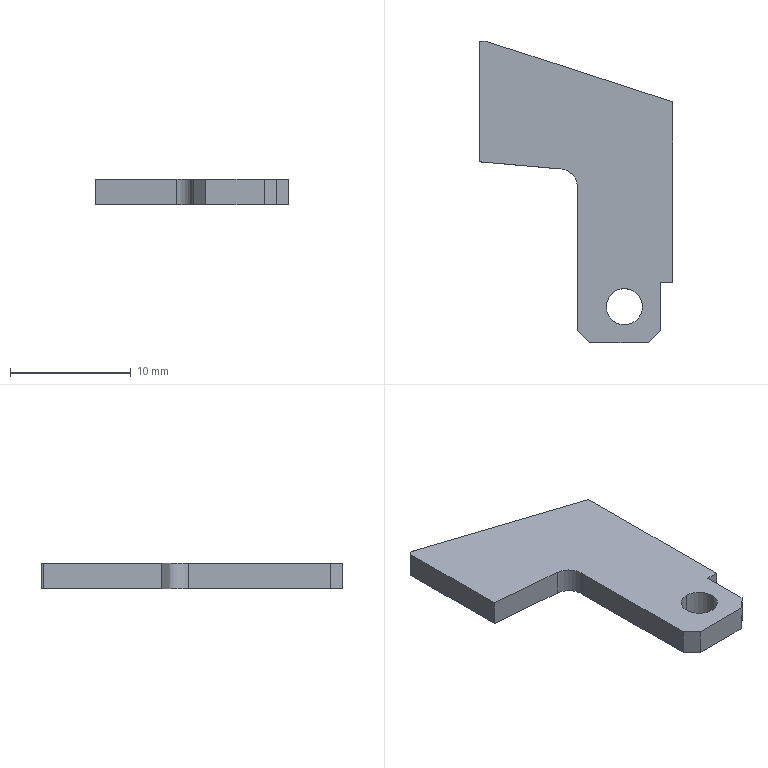Component | SolidWorks | 17268061-1 | 1 solid | 18 faces | box 16 x 25 x 2.1 mm | volume 482 mm3 | plane 13 | cylinder 5 | commonest cylinder face diameters 3 x3 0.4 x2 | material SKD-11 HRC58° Electroplated
STEP:
#1=CARTESIAN_POINT('',(2.264,-1.027,-0.3346));
#2=VERTEX_POINT('',#1);
#3=CARTESIAN_POINT('',(2.264,-1.145,-0.3346));
#4=VERTEX_POINT('',#3);
#5=CARTESIAN_POINT('',(2.264,-1.086,-0.3346));
#6=DIRECTION('',(-0.,0.,-1.));
#7=DIRECTION('',(0.,-1.,-0.));
#8=AXIS2_PLACEMENT_3D('',#5,#6,#7);
#9=CIRCLE('',#8,0.05906);
#10=EDGE_CURVE('',#2,#4,#9,.T.);
#11=ORIENTED_EDGE('',*,*,#10,.F.);
#12=CARTESIAN_POINT('',(2.264,-1.027,-0.4173));
#13=VERTEX_POINT('',#12);
#14=CARTESIAN_POINT('',(2.264,-1.027,-0.3346));
#15=DIRECTION('',(-0.,0.,-1.));
#16=VECTOR('',#15,39.37);
#17=LINE('',#14,#16);
#18=EDGE_CURVE('',#2,#13,#17,.T.);
#19=ORIENTED_EDGE('',*,*,#18,.T.);
#20=CARTESIAN_POINT('',(2.264,-1.145,-0.4173));
#21=VERTEX_POINT('',#20);
#22=CARTESIAN_POINT('',(2.264,-1.086,-0.4173));
#23=DIRECTION('',(-0.,0.,-1.));
#24=DIRECTION('',(0.,-1.,-0.));
#25=AXIS2_PLACEMENT_3D('',#22,#23,#24);
#26=CIRCLE('',#25,0.05906);
#27=EDGE_CURVE('',#13,#21,#26,.T.);
#28=ORIENTED_EDGE('',*,*,#27,.T.);
#29=CARTESIAN_POINT('',(2.264,-1.145,-0.3346));
#30=DIRECTION('',(-0.,0.,-1.));
#31=VECTOR('',#30,39.37);
#32=LINE('',#29,#31);
#33=EDGE_CURVE('',#4,#21,#32,.T.);
#34=ORIENTED_EDGE('',*,*,#33,.F.);
#35=EDGE_LOOP('',(#11,#19,#28,#34));
#36=FACE_OUTER_BOUND('',#35,.T.);
#37=CARTESIAN_POINT('',(2.264,-1.086,-0.3346));
#38=DIRECTION('',(-0.,0.,-1.));
#39=DIRECTION('',(0.,-1.,-0.));
#40=AXIS2_PLACEMENT_3D('',#37,#38,#39);
#41=CYLINDRICAL_SURFACE('',#40,0.05906);
#42=ADVANCED_FACE('',(#36),#41,.F.);
#43=CARTESIAN_POINT('',(2.421,-0.4179,-0.3346));
#44=VERTEX_POINT('',#43);
#45=CARTESIAN_POINT('',(2.421,-1.007,-0.3346));
#46=VERTEX_POINT('',#45);
#47=CARTESIAN_POINT('',(2.421,-0.2197,-0.3346));
#48=DIRECTION('',(-0.,-1.,-0.));
#49=VECTOR('',#48,39.37);
#50=LINE('',#47,#49);
#51=EDGE_CURVE('',#44,#46,#50,.T.);
#52=ORIENTED_EDGE('',*,*,#51,.T.);
#53=CARTESIAN_POINT('',(2.421,-1.007,-0.4173));
#54=VERTEX_POINT('',#53);
#55=CARTESIAN_POINT('',(2.421,-1.007,-0.3346));
#56=DIRECTION('',(-0.,0.,-1.));
#57=VECTOR('',#56,39.37);
#58=LINE('',#55,#57);
#59=EDGE_CURVE('',#46,#54,#58,.T.);
#60=ORIENTED_EDGE('',*,*,#59,.T.);
#61=CARTESIAN_POINT('',(2.421,-0.4179,-0.4173));
#62=VERTEX_POINT('',#61);
#63=CARTESIAN_POINT('',(2.421,-0.2197,-0.4173));
#64=DIRECTION('',(-0.,-1.,-0.));
#65=VECTOR('',#64,39.37);
#66=LINE('',#63,#65);
#67=EDGE_CURVE('',#62,#54,#66,.T.);
#68=ORIENTED_EDGE('',*,*,#67,.F.);
#69=CARTESIAN_POINT('',(2.421,-0.4179,-0.4173));
#70=DIRECTION('',(0.,-0.,1.));
#71=VECTOR('',#70,39.37);
#72=LINE('',#69,#71);
#73=EDGE_CURVE('',#62,#44,#72,.T.);
#74=ORIENTED_EDGE('',*,*,#73,.T.);
#75=EDGE_LOOP('',(#52,#60,#68,#74));
#76=FACE_OUTER_BOUND('',#75,.T.);
#77=CARTESIAN_POINT('',(2.421,-0.2197,-0.4173));
#78=DIRECTION('',(-1.,0.,0.));
#79=DIRECTION('',(0.,1.,0.));
#80=AXIS2_PLACEMENT_3D('',#77,#78,#79);
#81=PLANE('',#80);
#82=ADVANCED_FACE('',(#76),#81,.F.);
#83=CARTESIAN_POINT('',(2.343,-1.204,-0.3346));
#84=VERTEX_POINT('',#83);
#85=CARTESIAN_POINT('',(2.15,-1.204,-0.3346));
#86=VERTEX_POINT('',#85);
#87=CARTESIAN_POINT('',(2.421,-1.204,-0.3346));
#88=DIRECTION('',(-1.,0.,0.));
#89=VECTOR('',#88,39.37);
#90=LINE('',#87,#89);
#91=EDGE_CURVE('',#84,#86,#90,.T.);
#92=ORIENTED_EDGE('',*,*,#91,.T.);
#93=CARTESIAN_POINT('',(2.15,-1.204,-0.4173));
#94=VERTEX_POINT('',#93);
#95=CARTESIAN_POINT('',(2.15,-1.204,-0.4173));
#96=DIRECTION('',(-0.,0.,-1.));
#97=VECTOR('',#96,39.37);
#98=LINE('',#95,#97);
#99=EDGE_CURVE('',#86,#94,#98,.T.);
#100=ORIENTED_EDGE('',*,*,#99,.T.);
#101=CARTESIAN_POINT('',(2.343,-1.204,-0.4173));
#102=VERTEX_POINT('',#101);
#103=CARTESIAN_POINT('',(2.421,-1.204,-0.4173));
#104=DIRECTION('',(-1.,0.,0.));
#105=VECTOR('',#104,39.37);
#106=LINE('',#103,#105);
#107=EDGE_CURVE('',#102,#94,#106,.T.);
#108=ORIENTED_EDGE('',*,*,#107,.F.);
#109=CARTESIAN_POINT('',(2.343,-1.204,-0.4173));
#110=DIRECTION('',(0.,-0.,1.));
#111=VECTOR('',#110,39.37);
#112=LINE('',#109,#111);
#113=EDGE_CURVE('',#102,#84,#112,.T.);
#114=ORIENTED_EDGE('',*,*,#113,.T.);
#115=EDGE_LOOP('',(#92,#100,#108,#114));
#116=FACE_OUTER_BOUND('',#115,.T.);
#117=CARTESIAN_POINT('',(2.421,-1.204,-0.4173));
#118=DIRECTION('',(0.,1.,0.));
#119=DIRECTION('',(1.,-0.,-0.));
#120=AXIS2_PLACEMENT_3D('',#117,#118,#119);
#121=PLANE('',#120);
#122=ADVANCED_FACE('',(#116),#121,.F.);
#123=CARTESIAN_POINT('',(1.791,-0.6134,-0.3346));
#124=VERTEX_POINT('',#123);
#125=CARTESIAN_POINT('',(1.791,-0.2275,-0.3346));
#126=VERTEX_POINT('',#125);
#127=CARTESIAN_POINT('',(1.791,-0.2197,-0.3346));
#128=DIRECTION('',(0.,1.,0.));
#129=VECTOR('',#128,39.37);
#130=LINE('',#127,#129);
#131=EDGE_CURVE('',#124,#126,#130,.T.);
#132=ORIENTED_EDGE('',*,*,#131,.T.);
#133=CARTESIAN_POINT('',(1.791,-0.2275,-0.4173));
#134=VERTEX_POINT('',#133);
#135=CARTESIAN_POINT('',(1.791,-0.2275,-0.4173));
#136=DIRECTION('',(-0.,0.,-1.));
#137=VECTOR('',#136,39.37);
#138=LINE('',#135,#137);
#139=EDGE_CURVE('',#126,#134,#138,.T.);
#140=ORIENTED_EDGE('',*,*,#139,.T.);
#141=CARTESIAN_POINT('',(1.791,-0.6134,-0.4173));
#142=VERTEX_POINT('',#141);
#143=CARTESIAN_POINT('',(1.791,-0.2197,-0.4173));
#144=DIRECTION('',(0.,1.,0.));
#145=VECTOR('',#144,39.37);
#146=LINE('',#143,#145);
#147=EDGE_CURVE('',#142,#134,#146,.T.);
#148=ORIENTED_EDGE('',*,*,#147,.F.);
#149=CARTESIAN_POINT('',(1.791,-0.6134,-0.3346));
#150=DIRECTION('',(-0.,0.,-1.));
#151=VECTOR('',#150,39.37);
#152=LINE('',#149,#151);
#153=EDGE_CURVE('',#124,#142,#152,.T.);
#154=ORIENTED_EDGE('',*,*,#153,.F.);
#155=EDGE_LOOP('',(#132,#140,#148,#154));
#156=FACE_OUTER_BOUND('',#155,.T.);
#157=CARTESIAN_POINT('',(1.791,-0.2197,-0.4173));
#158=DIRECTION('',(1.,-0.,-0.));
#159=DIRECTION('',(-0.,-1.,-0.));
#160=AXIS2_PLACEMENT_3D('',#157,#158,#159);
#161=PLANE('',#160);
#162=ADVANCED_FACE('',(#156),#161,.F.);
#163=CARTESIAN_POINT('',(1.799,-0.2197,-0.3346));
#164=VERTEX_POINT('',#163);
#165=CARTESIAN_POINT('',(1.81,-0.2197,-0.3346));
#166=VERTEX_POINT('',#165);
#167=CARTESIAN_POINT('',(2.421,-0.2197,-0.3346));
#168=DIRECTION('',(1.,-0.,-0.));
#169=VECTOR('',#168,39.37);
#170=LINE('',#167,#169);
#171=EDGE_CURVE('',#164,#166,#170,.T.);
#172=ORIENTED_EDGE('',*,*,#171,.T.);
#173=CARTESIAN_POINT('',(1.81,-0.2197,-0.4173));
#174=VERTEX_POINT('',#173);
#175=CARTESIAN_POINT('',(1.81,-0.2197,-0.4173));
#176=DIRECTION('',(-0.,0.,-1.));
#177=VECTOR('',#176,39.37);
#178=LINE('',#175,#177);
#179=EDGE_CURVE('',#166,#174,#178,.T.);
#180=ORIENTED_EDGE('',*,*,#179,.T.);
#181=CARTESIAN_POINT('',(1.799,-0.2197,-0.4173));
#182=VERTEX_POINT('',#181);
#183=CARTESIAN_POINT('',(2.421,-0.2197,-0.4173));
#184=DIRECTION('',(1.,-0.,-0.));
#185=VECTOR('',#184,39.37);
#186=LINE('',#183,#185);
#187=EDGE_CURVE('',#182,#174,#186,.T.);
#188=ORIENTED_EDGE('',*,*,#187,.F.);
#189=CARTESIAN_POINT('',(1.799,-0.2197,-0.4173));
#190=DIRECTION('',(0.,-0.,1.));
#191=VECTOR('',#190,39.37);
#192=LINE('',#189,#191);
#193=EDGE_CURVE('',#182,#164,#192,.T.);
#194=ORIENTED_EDGE('',*,*,#193,.T.);
#195=EDGE_LOOP('',(#172,#180,#188,#194));
#196=FACE_OUTER_BOUND('',#195,.T.);
#197=CARTESIAN_POINT('',(2.421,-0.2197,-0.4173));
#198=DIRECTION('',(-0.,-1.,-0.));
#199=DIRECTION('',(-1.,0.,0.));
#200=AXIS2_PLACEMENT_3D('',#197,#198,#199);
#201=PLANE('',#200);
#202=ADVANCED_FACE('',(#196),#201,.F.);
#203=ORIENTED_EDGE('',*,*,#107,.T.);
#204=CARTESIAN_POINT('',(2.111,-1.165,-0.4173));
#205=VERTEX_POINT('',#204);
#206=CARTESIAN_POINT('',(2.286,-1.339,-0.4173));
#207=DIRECTION('',(-0.7071,0.7071,0.));
#208=VECTOR('',#207,39.37);
#209=LINE('',#206,#208);
#210=EDGE_CURVE('',#94,#205,#209,.T.);
#211=ORIENTED_EDGE('',*,*,#210,.T.);
#212=CARTESIAN_POINT('',(2.111,-0.7006,-0.4173));
#213=VERTEX_POINT('',#212);
#214=CARTESIAN_POINT('',(2.111,-0.7006,-0.4173));
#215=DIRECTION('',(-0.,-1.,-0.));
#216=VECTOR('',#215,39.37);
#217=LINE('',#214,#216);
#218=EDGE_CURVE('',#213,#205,#217,.T.);
#219=ORIENTED_EDGE('',*,*,#218,.F.);
#220=CARTESIAN_POINT('',(2.057,-0.6366,-0.4173));
#221=VERTEX_POINT('',#220);
#222=CARTESIAN_POINT('',(2.052,-0.6955,-0.4173));
#223=DIRECTION('',(0.,-0.,1.));
#224=DIRECTION('',(0.,-1.,-0.));
#225=AXIS2_PLACEMENT_3D('',#222,#223,#224);
#226=CIRCLE('',#225,0.05906);
#227=EDGE_CURVE('',#213,#221,#226,.T.);
#228=ORIENTED_EDGE('',*,*,#227,.T.);
#229=CARTESIAN_POINT('',(1.791,-0.6134,-0.4173));
#230=DIRECTION('',(0.9962,-0.08716,-0.));
#231=VECTOR('',#230,39.37);
#232=LINE('',#229,#231);
#233=EDGE_CURVE('',#142,#221,#232,.T.);
#234=ORIENTED_EDGE('',*,*,#233,.F.);
#235=ORIENTED_EDGE('',*,*,#147,.T.);
#236=CARTESIAN_POINT('',(1.799,-0.2275,-0.4173));
#237=DIRECTION('',(-0.,0.,-1.));
#238=DIRECTION('',(0.,-1.,0.));
#239=AXIS2_PLACEMENT_3D('',#236,#237,#238);
#240=CIRCLE('',#239,0.007874);
#241=EDGE_CURVE('',#134,#182,#240,.T.);
#242=ORIENTED_EDGE('',*,*,#241,.T.);
#243=ORIENTED_EDGE('',*,*,#187,.T.);
#244=CARTESIAN_POINT('',(1.812,-0.22,-0.4173));
#245=VERTEX_POINT('',#244);
#246=CARTESIAN_POINT('',(1.81,-0.2275,-0.4173));
#247=DIRECTION('',(-0.,0.,-1.));
#248=DIRECTION('',(0.,-1.,0.));
#249=AXIS2_PLACEMENT_3D('',#246,#247,#248);
#250=CIRCLE('',#249,0.007874);
#251=EDGE_CURVE('',#174,#245,#250,.T.);
#252=ORIENTED_EDGE('',*,*,#251,.T.);
#253=CARTESIAN_POINT('',(2.421,-0.4179,-0.4173));
#254=DIRECTION('',(0.9511,-0.309,-0.));
#255=VECTOR('',#254,39.37);
#256=LINE('',#253,#255);
#257=EDGE_CURVE('',#245,#62,#256,.T.);
#258=ORIENTED_EDGE('',*,*,#257,.T.);
#259=ORIENTED_EDGE('',*,*,#67,.T.);
#260=CARTESIAN_POINT('',(2.382,-1.007,-0.4173));
#261=VERTEX_POINT('',#260);
#262=CARTESIAN_POINT('',(2.421,-1.007,-0.4173));
#263=DIRECTION('',(1.,-0.,-0.));
#264=VECTOR('',#263,39.37);
#265=LINE('',#262,#264);
#266=EDGE_CURVE('',#261,#54,#265,.T.);
#267=ORIENTED_EDGE('',*,*,#266,.F.);
#268=CARTESIAN_POINT('',(2.382,-1.165,-0.4173));
#269=VERTEX_POINT('',#268);
#270=CARTESIAN_POINT('',(2.382,-1.007,-0.4173));
#271=DIRECTION('',(0.,1.,0.));
#272=VECTOR('',#271,39.37);
#273=LINE('',#270,#272);
#274=EDGE_CURVE('',#269,#261,#273,.T.);
#275=ORIENTED_EDGE('',*,*,#274,.F.);
#276=CARTESIAN_POINT('',(2.382,-1.165,-0.4173));
#277=DIRECTION('',(-0.7071,-0.7071,0.));
#278=VECTOR('',#277,39.37);
#279=LINE('',#276,#278);
#280=EDGE_CURVE('',#269,#102,#279,.T.);
#281=ORIENTED_EDGE('',*,*,#280,.T.);
#282=EDGE_LOOP('',(#203,#211,#219,#228,#234,#235,#242,#243,#252,#258,#259,#267,#275,#281));
#283=FACE_OUTER_BOUND('',#282,.T.);
#284=CARTESIAN_POINT('',(2.264,-1.086,-0.4173));
#285=DIRECTION('',(-0.,0.,-1.));
#286=DIRECTION('',(0.,-1.,-0.));
#287=AXIS2_PLACEMENT_3D('',#284,#285,#286);
#288=CIRCLE('',#287,0.05906);
#289=EDGE_CURVE('',#21,#13,#288,.T.);
#290=ORIENTED_EDGE('',*,*,#289,.F.);
#291=ORIENTED_EDGE('',*,*,#27,.F.);
#292=EDGE_LOOP('',(#290,#291));
#293=FACE_BOUND('',#292,.T.);
#294=CARTESIAN_POINT('',(2.421,-1.204,-0.4173));
#295=DIRECTION('',(-0.,0.,-1.));
#296=DIRECTION('',(-0.,-1.,-0.));
#297=AXIS2_PLACEMENT_3D('',#294,#295,#296);
#298=PLANE('',#297);
#299=ADVANCED_FACE('',(#283,#293),#298,.T.);
#300=CARTESIAN_POINT('',(2.264,-1.086,-0.3346));
#301=DIRECTION('',(-0.,0.,-1.));
#302=DIRECTION('',(0.,-1.,-0.));
#303=AXIS2_PLACEMENT_3D('',#300,#301,#302);
#304=CIRCLE('',#303,0.05906);
#305=EDGE_CURVE('',#4,#2,#304,.T.);
#306=ORIENTED_EDGE('',*,*,#305,.T.);
#307=ORIENTED_EDGE('',*,*,#10,.T.);
#308=EDGE_LOOP('',(#306,#307));
#309=FACE_BOUND('',#308,.T.);
#310=CARTESIAN_POINT('',(2.111,-0.7006,-0.3346));
#311=VERTEX_POINT('',#310);
#312=CARTESIAN_POINT('',(2.111,-1.165,-0.3346));
#313=VERTEX_POINT('',#312);
#314=CARTESIAN_POINT('',(2.111,-0.7006,-0.3346));
#315=DIRECTION('',(-0.,-1.,-0.));
#316=VECTOR('',#315,39.37);
#317=LINE('',#314,#316);
#318=EDGE_CURVE('',#311,#313,#317,.T.);
#319=ORIENTED_EDGE('',*,*,#318,.T.);
#320=CARTESIAN_POINT('',(2.15,-1.204,-0.3346));
#321=DIRECTION('',(0.7071,-0.7071,-0.));
#322=VECTOR('',#321,39.37);
#323=LINE('',#320,#322);
#324=EDGE_CURVE('',#313,#86,#323,.T.);
#325=ORIENTED_EDGE('',*,*,#324,.T.);
#326=ORIENTED_EDGE('',*,*,#91,.F.);
#327=CARTESIAN_POINT('',(2.382,-1.165,-0.3346));
#328=VERTEX_POINT('',#327);
#329=CARTESIAN_POINT('',(2.382,-1.165,-0.3346));
#330=DIRECTION('',(0.7071,0.7071,-0.));
#331=VECTOR('',#330,39.37);
#332=LINE('',#329,#331);
#333=EDGE_CURVE('',#84,#328,#332,.T.);
#334=ORIENTED_EDGE('',*,*,#333,.T.);
#335=CARTESIAN_POINT('',(2.382,-1.007,-0.3346));
#336=VERTEX_POINT('',#335);
#337=CARTESIAN_POINT('',(2.382,-1.007,-0.3346));
#338=DIRECTION('',(0.,1.,0.));
#339=VECTOR('',#338,39.37);
#340=LINE('',#337,#339);
#341=EDGE_CURVE('',#328,#336,#340,.T.);
#342=ORIENTED_EDGE('',*,*,#341,.T.);
#343=CARTESIAN_POINT('',(2.421,-1.007,-0.3346));
#344=DIRECTION('',(1.,-0.,-0.));
#345=VECTOR('',#344,39.37);
#346=LINE('',#343,#345);
#347=EDGE_CURVE('',#336,#46,#346,.T.);
#348=ORIENTED_EDGE('',*,*,#347,.T.);
#349=ORIENTED_EDGE('',*,*,#51,.F.);
#350=CARTESIAN_POINT('',(1.812,-0.22,-0.3346));
#351=VERTEX_POINT('',#350);
#352=CARTESIAN_POINT('',(2.421,-0.4179,-0.3346));
#353=DIRECTION('',(0.9511,-0.309,-0.));
#354=VECTOR('',#353,39.37);
#355=LINE('',#352,#354);
#356=EDGE_CURVE('',#351,#44,#355,.T.);
#357=ORIENTED_EDGE('',*,*,#356,.F.);
#358=CARTESIAN_POINT('',(1.81,-0.2275,-0.3346));
#359=DIRECTION('',(0.,-0.,1.));
#360=DIRECTION('',(0.,-1.,0.));
#361=AXIS2_PLACEMENT_3D('',#358,#359,#360);
#362=CIRCLE('',#361,0.007874);
#363=EDGE_CURVE('',#351,#166,#362,.T.);
#364=ORIENTED_EDGE('',*,*,#363,.T.);
#365=ORIENTED_EDGE('',*,*,#171,.F.);
#366=CARTESIAN_POINT('',(1.799,-0.2275,-0.3346));
#367=DIRECTION('',(0.,-0.,1.));
#368=DIRECTION('',(0.,-1.,0.));
#369=AXIS2_PLACEMENT_3D('',#366,#367,#368);
#370=CIRCLE('',#369,0.007874);
#371=EDGE_CURVE('',#164,#126,#370,.T.);
#372=ORIENTED_EDGE('',*,*,#371,.T.);
#373=ORIENTED_EDGE('',*,*,#131,.F.);
#374=CARTESIAN_POINT('',(2.057,-0.6366,-0.3346));
#375=VERTEX_POINT('',#374);
#376=CARTESIAN_POINT('',(1.791,-0.6134,-0.3346));
#377=DIRECTION('',(0.9962,-0.08716,-0.));
#378=VECTOR('',#377,39.37);
#379=LINE('',#376,#378);
#380=EDGE_CURVE('',#124,#375,#379,.T.);
#381=ORIENTED_EDGE('',*,*,#380,.T.);
#382=CARTESIAN_POINT('',(2.052,-0.6955,-0.3346));
#383=DIRECTION('',(-0.,0.,-1.));
#384=DIRECTION('',(0.,-1.,-0.));
#385=AXIS2_PLACEMENT_3D('',#382,#383,#384);
#386=CIRCLE('',#385,0.05906);
#387=EDGE_CURVE('',#375,#311,#386,.T.);
#388=ORIENTED_EDGE('',*,*,#387,.T.);
#389=EDGE_LOOP('',(#319,#325,#326,#334,#342,#348,#349,#357,#364,#365,#372,#373,#381,#388));
#390=FACE_OUTER_BOUND('',#389,.T.);
#391=CARTESIAN_POINT('',(2.421,-1.204,-0.3346));
#392=DIRECTION('',(-0.,0.,-1.));
#393=DIRECTION('',(-0.,-1.,-0.));
#394=AXIS2_PLACEMENT_3D('',#391,#392,#393);
#395=PLANE('',#394);
#396=ADVANCED_FACE('',(#309,#390),#395,.F.);
#397=ORIENTED_EDGE('',*,*,#18,.F.);
#398=ORIENTED_EDGE('',*,*,#305,.F.);
#399=ORIENTED_EDGE('',*,*,#33,.T.);
#400=ORIENTED_EDGE('',*,*,#289,.T.);
#401=EDGE_LOOP('',(#397,#398,#399,#400));
#402=FACE_OUTER_BOUND('',#401,.T.);
#403=CARTESIAN_POINT('',(2.264,-1.086,-0.3346));
#404=DIRECTION('',(-0.,0.,-1.));
#405=DIRECTION('',(0.,-1.,-0.));
#406=AXIS2_PLACEMENT_3D('',#403,#404,#405);
#407=CYLINDRICAL_SURFACE('',#406,0.05906);
#408=ADVANCED_FACE('',(#402),#407,.F.);
#409=ORIENTED_EDGE('',*,*,#233,.T.);
#410=CARTESIAN_POINT('',(2.057,-0.6366,-0.3346));
#411=DIRECTION('',(0.,-0.,1.));
#412=VECTOR('',#411,39.37);
#413=LINE('',#410,#412);
#414=EDGE_CURVE('',#221,#375,#413,.T.);
#415=ORIENTED_EDGE('',*,*,#414,.T.);
#416=ORIENTED_EDGE('',*,*,#380,.F.);
#417=ORIENTED_EDGE('',*,*,#153,.T.);
#418=EDGE_LOOP('',(#409,#415,#416,#417));
#419=FACE_OUTER_BOUND('',#418,.T.);
#420=CARTESIAN_POINT('',(1.791,-0.6134,-0.3346));
#421=DIRECTION('',(0.08716,0.9962,0.));
#422=DIRECTION('',(0.9962,-0.08716,-0.));
#423=AXIS2_PLACEMENT_3D('',#420,#421,#422);
#424=PLANE('',#423);
#425=ADVANCED_FACE('',(#419),#424,.F.);
#426=ORIENTED_EDGE('',*,*,#257,.F.);
#427=CARTESIAN_POINT('',(1.812,-0.22,-0.4173));
#428=DIRECTION('',(0.,-0.,1.));
#429=VECTOR('',#428,39.37);
#430=LINE('',#427,#429);
#431=EDGE_CURVE('',#245,#351,#430,.T.);
#432=ORIENTED_EDGE('',*,*,#431,.T.);
#433=ORIENTED_EDGE('',*,*,#356,.T.);
#434=ORIENTED_EDGE('',*,*,#73,.F.);
#435=EDGE_LOOP('',(#426,#432,#433,#434));
#436=FACE_OUTER_BOUND('',#435,.T.);
#437=CARTESIAN_POINT('',(2.421,-0.4179,-0.4173));
#438=DIRECTION('',(-0.309,-0.9511,-0.));
#439=DIRECTION('',(-0.9511,0.309,0.));
#440=AXIS2_PLACEMENT_3D('',#437,#438,#439);
#441=PLANE('',#440);
#442=ADVANCED_FACE('',(#436),#441,.F.);
#443=ORIENTED_EDGE('',*,*,#251,.F.);
#444=ORIENTED_EDGE('',*,*,#179,.F.);
#445=ORIENTED_EDGE('',*,*,#363,.F.);
#446=ORIENTED_EDGE('',*,*,#431,.F.);
#447=EDGE_LOOP('',(#443,#444,#445,#446));
#448=FACE_OUTER_BOUND('',#447,.T.);
#449=CARTESIAN_POINT('',(1.81,-0.2275,-0.4173));
#450=DIRECTION('',(0.,-0.,1.));
#451=DIRECTION('',(0.,1.,0.));
#452=AXIS2_PLACEMENT_3D('',#449,#450,#451);
#453=CYLINDRICAL_SURFACE('',#452,0.007874);
#454=ADVANCED_FACE('',(#448),#453,.T.);
#455=ORIENTED_EDGE('',*,*,#241,.F.);
#456=ORIENTED_EDGE('',*,*,#139,.F.);
#457=ORIENTED_EDGE('',*,*,#371,.F.);
#458=ORIENTED_EDGE('',*,*,#193,.F.);
#459=EDGE_LOOP('',(#455,#456,#457,#458));
#460=FACE_OUTER_BOUND('',#459,.T.);
#461=CARTESIAN_POINT('',(1.799,-0.2275,-0.4173));
#462=DIRECTION('',(0.,-0.,1.));
#463=DIRECTION('',(0.,1.,0.));
#464=AXIS2_PLACEMENT_3D('',#461,#462,#463);
#465=CYLINDRICAL_SURFACE('',#464,0.007874);
#466=ADVANCED_FACE('',(#460),#465,.T.);
#467=ORIENTED_EDGE('',*,*,#266,.T.);
#468=ORIENTED_EDGE('',*,*,#59,.F.);
#469=ORIENTED_EDGE('',*,*,#347,.F.);
#470=CARTESIAN_POINT('',(2.382,-1.007,-0.3346));
#471=DIRECTION('',(-0.,0.,-1.));
#472=VECTOR('',#471,39.37);
#473=LINE('',#470,#472);
#474=EDGE_CURVE('',#336,#261,#473,.T.);
#475=ORIENTED_EDGE('',*,*,#474,.T.);
#476=EDGE_LOOP('',(#467,#468,#469,#475));
#477=FACE_OUTER_BOUND('',#476,.T.);
#478=CARTESIAN_POINT('',(2.421,-1.007,-0.3346));
#479=DIRECTION('',(0.,1.,0.));
#480=DIRECTION('',(1.,-0.,-0.));
#481=AXIS2_PLACEMENT_3D('',#478,#479,#480);
#482=PLANE('',#481);
#483=ADVANCED_FACE('',(#477),#482,.F.);
#484=ORIENTED_EDGE('',*,*,#341,.F.);
#485=CARTESIAN_POINT('',(2.382,-1.165,-0.3346));
#486=DIRECTION('',(-0.,0.,-1.));
#487=VECTOR('',#486,39.37);
#488=LINE('',#485,#487);
#489=EDGE_CURVE('',#328,#269,#488,.T.);
#490=ORIENTED_EDGE('',*,*,#489,.T.);
#491=ORIENTED_EDGE('',*,*,#274,.T.);
#492=ORIENTED_EDGE('',*,*,#474,.F.);
#493=EDGE_LOOP('',(#484,#490,#491,#492));
#494=FACE_OUTER_BOUND('',#493,.T.);
#495=CARTESIAN_POINT('',(2.382,-1.007,-0.3346));
#496=DIRECTION('',(-1.,0.,0.));
#497=DIRECTION('',(0.,1.,0.));
#498=AXIS2_PLACEMENT_3D('',#495,#496,#497);
#499=PLANE('',#498);
#500=ADVANCED_FACE('',(#494),#499,.F.);
#501=ORIENTED_EDGE('',*,*,#387,.F.);
#502=ORIENTED_EDGE('',*,*,#414,.F.);
#503=ORIENTED_EDGE('',*,*,#227,.F.);
#504=CARTESIAN_POINT('',(2.111,-0.7006,-0.4173));
#505=DIRECTION('',(-0.,0.,-1.));
#506=VECTOR('',#505,39.37);
#507=LINE('',#504,#506);
#508=EDGE_CURVE('',#311,#213,#507,.T.);
#509=ORIENTED_EDGE('',*,*,#508,.F.);
#510=EDGE_LOOP('',(#501,#502,#503,#509));
#511=FACE_OUTER_BOUND('',#510,.T.);
#512=CARTESIAN_POINT('',(2.052,-0.6955,-0.3346));
#513=DIRECTION('',(0.,-0.,1.));
#514=DIRECTION('',(0.,1.,0.));
#515=AXIS2_PLACEMENT_3D('',#512,#513,#514);
#516=CYLINDRICAL_SURFACE('',#515,0.05906);
#517=ADVANCED_FACE('',(#511),#516,.F.);
#518=ORIENTED_EDGE('',*,*,#218,.T.);
#519=CARTESIAN_POINT('',(2.111,-1.165,-0.3346));
#520=DIRECTION('',(0.,-0.,1.));
#521=VECTOR('',#520,39.37);
#522=LINE('',#519,#521);
#523=EDGE_CURVE('',#205,#313,#522,.T.);
#524=ORIENTED_EDGE('',*,*,#523,.T.);
#525=ORIENTED_EDGE('',*,*,#318,.F.);
#526=ORIENTED_EDGE('',*,*,#508,.T.);
#527=EDGE_LOOP('',(#518,#524,#525,#526));
#528=FACE_OUTER_BOUND('',#527,.T.);
#529=CARTESIAN_POINT('',(2.111,-0.7006,-0.3346));
#530=DIRECTION('',(1.,-0.,-0.));
#531=DIRECTION('',(-0.,-1.,-0.));
#532=AXIS2_PLACEMENT_3D('',#529,#530,#531);
#533=PLANE('',#532);
#534=ADVANCED_FACE('',(#528),#533,.F.);
#535=ORIENTED_EDGE('',*,*,#324,.F.);
#536=ORIENTED_EDGE('',*,*,#523,.F.);
#537=ORIENTED_EDGE('',*,*,#210,.F.);
#538=ORIENTED_EDGE('',*,*,#99,.F.);
#539=EDGE_LOOP('',(#535,#536,#537,#538));
#540=FACE_OUTER_BOUND('',#539,.T.);
#541=CARTESIAN_POINT('',(2.15,-1.204,-0.4173));
#542=DIRECTION('',(0.7071,0.7071,-0.));
#543=DIRECTION('',(-0.,0.,-1.));
#544=AXIS2_PLACEMENT_3D('',#541,#542,#543);
#545=PLANE('',#544);
#546=ADVANCED_FACE('',(#540),#545,.F.);
#547=ORIENTED_EDGE('',*,*,#333,.F.);
#548=ORIENTED_EDGE('',*,*,#113,.F.);
#549=ORIENTED_EDGE('',*,*,#280,.F.);
#550=ORIENTED_EDGE('',*,*,#489,.F.);
#551=EDGE_LOOP('',(#547,#548,#549,#550));
#552=FACE_OUTER_BOUND('',#551,.T.);
#553=CARTESIAN_POINT('',(2.382,-1.165,-0.3346));
#554=DIRECTION('',(-0.7071,0.7071,0.));
#555=DIRECTION('',(-0.,0.,-1.));
#556=AXIS2_PLACEMENT_3D('',#553,#554,#555);
#557=PLANE('',#556);
#558=ADVANCED_FACE('',(#552),#557,.F.);
#559=CLOSED_SHELL('',(#42,#82,#122,#162,#202,#299,#396,#408,#425,#442,#454,#466,#483,#500,#517,#534,#546,#558));
#560=MANIFOLD_SOLID_BREP('',#559);
#561=CARTESIAN_POINT('',(0.,0.,0.));
#562=DIRECTION('',(0.,0.,1.));
#563=DIRECTION('',(1.,0.,0.));
#564=AXIS2_PLACEMENT_3D('',#561,#562,#563);
#565=(LENGTH_UNIT()NAMED_UNIT(*)SI_UNIT($,.METRE.));
#566=LENGTH_MEASURE_WITH_UNIT(LENGTH_MEASURE(0.0254),#565);
#567=DIMENSIONAL_EXPONENTS(1.,0.,0.,0.,0.,0.,0.);
#568=(CONVERSION_BASED_UNIT('',#566)LENGTH_UNIT()NAMED_UNIT(#567));
#569=UNCERTAINTY_MEASURE_WITH_UNIT(LENGTH_MEASURE(0.00001),#568,'','');
#570=(NAMED_UNIT(*)PLANE_ANGLE_UNIT()SI_UNIT($,.RADIAN.));
#571=(NAMED_UNIT(*)SI_UNIT($,.STERADIAN.)SOLID_ANGLE_UNIT());
#572=(GEOMETRIC_REPRESENTATION_CONTEXT(3)GLOBAL_UNCERTAINTY_ASSIGNED_CONTEXT((#569))GLOBAL_UNIT_ASSIGNED_CONTEXT((#568,#570,#571))REPRESENTATION_CONTEXT('',''));
#573=ADVANCED_BREP_SHAPE_REPRESENTATION('',(#560,#564),#572);
#574=COLOUR_RGB('',0.7922,0.8196,0.9333);
#575=FILL_AREA_STYLE_COLOUR('',#574);
#576=FILL_AREA_STYLE('',(#575));
#577=SURFACE_STYLE_FILL_AREA(#576);
#578=SURFACE_SIDE_STYLE('',(#577));
#579=SURFACE_STYLE_USAGE(.BOTH.,#578);
#580=PRESENTATION_STYLE_ASSIGNMENT((#579));
#581=STYLED_ITEM('',(#580),#560);
#582=(LENGTH_UNIT()NAMED_UNIT(*)SI_UNIT($,.METRE.));
#583=LENGTH_MEASURE_WITH_UNIT(LENGTH_MEASURE(0.0254),#582);
#584=DIMENSIONAL_EXPONENTS(1.,0.,0.,0.,0.,0.,0.);
#585=(CONVERSION_BASED_UNIT('',#583)LENGTH_UNIT()NAMED_UNIT(#584));
#586=UNCERTAINTY_MEASURE_WITH_UNIT(LENGTH_MEASURE(0.00001),#585,'','');
#587=(NAMED_UNIT(*)PLANE_ANGLE_UNIT()SI_UNIT($,.RADIAN.));
#588=(NAMED_UNIT(*)SI_UNIT($,.STERADIAN.)SOLID_ANGLE_UNIT());
#589=(GEOMETRIC_REPRESENTATION_CONTEXT(3)GLOBAL_UNCERTAINTY_ASSIGNED_CONTEXT((#586))GLOBAL_UNIT_ASSIGNED_CONTEXT((#585,#587,#588))REPRESENTATION_CONTEXT('',''));
#590=MECHANICAL_DESIGN_GEOMETRIC_PRESENTATION_REPRESENTATION('',(#581),#589);
#591=PRESENTATION_LAYER_ASSIGNMENT('','',(#581));